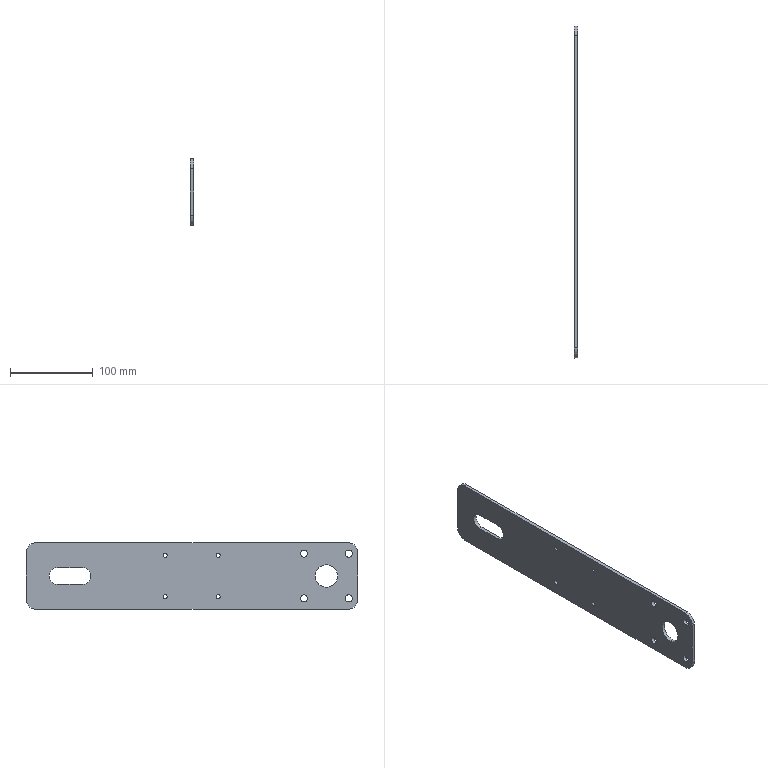Component | SolidWorks | BeltLineSidePlate-3_YL1.sldasm-Part-90-1 | 1 solid | 32 faces | box 4 x 400 x 80 mm | volume 120337 mm3 | cylinder 24 | plane 8 | commonest cylinder face diameters 5 x8 8.5 x8 24 x4 27 x2 20 x2
STEP:
#1=CARTESIAN_POINT('',(227.52,115.275,0.7825));
#2=VERTEX_POINT('',#1);
#3=CARTESIAN_POINT('',(227.52,115.275,0.9793));
#4=VERTEX_POINT('',#3);
#5=CARTESIAN_POINT('',(227.52,115.275,0.8809));
#6=DIRECTION('',(-1.,-0.,-0.));
#7=DIRECTION('',(0.,0.,1.));
#8=AXIS2_PLACEMENT_3D('',#5,#6,#7);
#9=CIRCLE('',#8,0.09843);
#10=EDGE_CURVE('',#2,#4,#9,.T.);
#11=ORIENTED_EDGE('',*,*,#10,.F.);
#12=CARTESIAN_POINT('',(227.362,115.275,0.7825));
#13=VERTEX_POINT('',#12);
#14=CARTESIAN_POINT('',(227.205,115.275,0.7825));
#15=DIRECTION('',(-1.,-0.,-0.));
#16=VECTOR('',#15,39.37);
#17=LINE('',#14,#16);
#18=EDGE_CURVE('',#2,#13,#17,.T.);
#19=ORIENTED_EDGE('',*,*,#18,.T.);
#20=CARTESIAN_POINT('',(227.362,115.275,0.9793));
#21=VERTEX_POINT('',#20);
#22=CARTESIAN_POINT('',(227.362,115.275,0.8809));
#23=DIRECTION('',(1.,0.,-0.));
#24=DIRECTION('',(0.,-1.,0.));
#25=AXIS2_PLACEMENT_3D('',#22,#23,#24);
#26=CIRCLE('',#25,0.09843);
#27=EDGE_CURVE('',#21,#13,#26,.T.);
#28=ORIENTED_EDGE('',*,*,#27,.F.);
#29=CARTESIAN_POINT('',(227.205,115.275,0.9793));
#30=DIRECTION('',(-1.,-0.,-0.));
#31=VECTOR('',#30,39.37);
#32=LINE('',#29,#31);
#33=EDGE_CURVE('',#4,#21,#32,.T.);
#34=ORIENTED_EDGE('',*,*,#33,.F.);
#35=EDGE_LOOP('',(#11,#19,#28,#34));
#36=FACE_OUTER_BOUND('',#35,.T.);
#37=CARTESIAN_POINT('',(227.205,115.275,0.8809));
#38=DIRECTION('',(-1.,-0.,-0.));
#39=DIRECTION('',(0.,0.,1.));
#40=AXIS2_PLACEMENT_3D('',#37,#38,#39);
#41=CYLINDRICAL_SURFACE('',#40,0.09843);
#42=ADVANCED_FACE('',(#36),#41,.F.);
#43=CARTESIAN_POINT('',(227.52,115.275,2.751));
#44=VERTEX_POINT('',#43);
#45=CARTESIAN_POINT('',(227.52,115.275,2.948));
#46=VERTEX_POINT('',#45);
#47=CARTESIAN_POINT('',(227.52,115.275,2.849));
#48=DIRECTION('',(-1.,-0.,-0.));
#49=DIRECTION('',(0.,0.,1.));
#50=AXIS2_PLACEMENT_3D('',#47,#48,#49);
#51=CIRCLE('',#50,0.09843);
#52=EDGE_CURVE('',#44,#46,#51,.T.);
#53=ORIENTED_EDGE('',*,*,#52,.F.);
#54=CARTESIAN_POINT('',(227.362,115.275,2.751));
#55=VERTEX_POINT('',#54);
#56=CARTESIAN_POINT('',(227.205,115.275,2.751));
#57=DIRECTION('',(-1.,-0.,-0.));
#58=VECTOR('',#57,39.37);
#59=LINE('',#56,#58);
#60=EDGE_CURVE('',#44,#55,#59,.T.);
#61=ORIENTED_EDGE('',*,*,#60,.T.);
#62=CARTESIAN_POINT('',(227.362,115.275,2.948));
#63=VERTEX_POINT('',#62);
#64=CARTESIAN_POINT('',(227.362,115.275,2.849));
#65=DIRECTION('',(1.,0.,-0.));
#66=DIRECTION('',(0.,-1.,0.));
#67=AXIS2_PLACEMENT_3D('',#64,#65,#66);
#68=CIRCLE('',#67,0.09843);
#69=EDGE_CURVE('',#63,#55,#68,.T.);
#70=ORIENTED_EDGE('',*,*,#69,.F.);
#71=CARTESIAN_POINT('',(227.205,115.275,2.948));
#72=DIRECTION('',(-1.,-0.,-0.));
#73=VECTOR('',#72,39.37);
#74=LINE('',#71,#73);
#75=EDGE_CURVE('',#46,#63,#74,.T.);
#76=ORIENTED_EDGE('',*,*,#75,.F.);
#77=EDGE_LOOP('',(#53,#61,#70,#76));
#78=FACE_OUTER_BOUND('',#77,.T.);
#79=CARTESIAN_POINT('',(227.205,115.275,2.849));
#80=DIRECTION('',(-1.,-0.,-0.));
#81=DIRECTION('',(0.,0.,1.));
#82=AXIS2_PLACEMENT_3D('',#79,#80,#81);
#83=CYLINDRICAL_SURFACE('',#82,0.09843);
#84=ADVANCED_FACE('',(#78),#83,.F.);
#85=CARTESIAN_POINT('',(227.52,112.756,0.7825));
#86=VERTEX_POINT('',#85);
#87=CARTESIAN_POINT('',(227.52,112.756,0.9793));
#88=VERTEX_POINT('',#87);
#89=CARTESIAN_POINT('',(227.52,112.756,0.8809));
#90=DIRECTION('',(-1.,-0.,-0.));
#91=DIRECTION('',(0.,0.,1.));
#92=AXIS2_PLACEMENT_3D('',#89,#90,#91);
#93=CIRCLE('',#92,0.09843);
#94=EDGE_CURVE('',#86,#88,#93,.T.);
#95=ORIENTED_EDGE('',*,*,#94,.F.);
#96=CARTESIAN_POINT('',(227.362,112.756,0.7825));
#97=VERTEX_POINT('',#96);
#98=CARTESIAN_POINT('',(227.205,112.756,0.7825));
#99=DIRECTION('',(-1.,-0.,-0.));
#100=VECTOR('',#99,39.37);
#101=LINE('',#98,#100);
#102=EDGE_CURVE('',#86,#97,#101,.T.);
#103=ORIENTED_EDGE('',*,*,#102,.T.);
#104=CARTESIAN_POINT('',(227.362,112.756,0.9793));
#105=VERTEX_POINT('',#104);
#106=CARTESIAN_POINT('',(227.362,112.756,0.8809));
#107=DIRECTION('',(1.,0.,-0.));
#108=DIRECTION('',(0.,-1.,0.));
#109=AXIS2_PLACEMENT_3D('',#106,#107,#108);
#110=CIRCLE('',#109,0.09843);
#111=EDGE_CURVE('',#105,#97,#110,.T.);
#112=ORIENTED_EDGE('',*,*,#111,.F.);
#113=CARTESIAN_POINT('',(227.205,112.756,0.9793));
#114=DIRECTION('',(-1.,-0.,-0.));
#115=VECTOR('',#114,39.37);
#116=LINE('',#113,#115);
#117=EDGE_CURVE('',#88,#105,#116,.T.);
#118=ORIENTED_EDGE('',*,*,#117,.F.);
#119=EDGE_LOOP('',(#95,#103,#112,#118));
#120=FACE_OUTER_BOUND('',#119,.T.);
#121=CARTESIAN_POINT('',(227.205,112.756,0.8809));
#122=DIRECTION('',(-1.,-0.,-0.));
#123=DIRECTION('',(0.,0.,1.));
#124=AXIS2_PLACEMENT_3D('',#121,#122,#123);
#125=CYLINDRICAL_SURFACE('',#124,0.09843);
#126=ADVANCED_FACE('',(#120),#125,.F.);
#127=CARTESIAN_POINT('',(227.52,112.756,2.751));
#128=VERTEX_POINT('',#127);
#129=CARTESIAN_POINT('',(227.52,112.756,2.948));
#130=VERTEX_POINT('',#129);
#131=CARTESIAN_POINT('',(227.52,112.756,2.849));
#132=DIRECTION('',(-1.,-0.,-0.));
#133=DIRECTION('',(0.,0.,1.));
#134=AXIS2_PLACEMENT_3D('',#131,#132,#133);
#135=CIRCLE('',#134,0.09843);
#136=EDGE_CURVE('',#128,#130,#135,.T.);
#137=ORIENTED_EDGE('',*,*,#136,.F.);
#138=CARTESIAN_POINT('',(227.362,112.756,2.751));
#139=VERTEX_POINT('',#138);
#140=CARTESIAN_POINT('',(227.205,112.756,2.751));
#141=DIRECTION('',(-1.,-0.,-0.));
#142=VECTOR('',#141,39.37);
#143=LINE('',#140,#142);
#144=EDGE_CURVE('',#128,#139,#143,.T.);
#145=ORIENTED_EDGE('',*,*,#144,.T.);
#146=CARTESIAN_POINT('',(227.362,112.756,2.948));
#147=VERTEX_POINT('',#146);
#148=CARTESIAN_POINT('',(227.362,112.756,2.849));
#149=DIRECTION('',(1.,0.,-0.));
#150=DIRECTION('',(0.,-1.,0.));
#151=AXIS2_PLACEMENT_3D('',#148,#149,#150);
#152=CIRCLE('',#151,0.09843);
#153=EDGE_CURVE('',#147,#139,#152,.T.);
#154=ORIENTED_EDGE('',*,*,#153,.F.);
#155=CARTESIAN_POINT('',(227.205,112.756,2.948));
#156=DIRECTION('',(-1.,-0.,-0.));
#157=VECTOR('',#156,39.37);
#158=LINE('',#155,#157);
#159=EDGE_CURVE('',#130,#147,#158,.T.);
#160=ORIENTED_EDGE('',*,*,#159,.F.);
#161=EDGE_LOOP('',(#137,#145,#154,#160));
#162=FACE_OUTER_BOUND('',#161,.T.);
#163=CARTESIAN_POINT('',(227.205,112.756,2.849));
#164=DIRECTION('',(-1.,-0.,-0.));
#165=DIRECTION('',(0.,0.,1.));
#166=AXIS2_PLACEMENT_3D('',#163,#164,#165);
#167=CYLINDRICAL_SURFACE('',#166,0.09843);
#168=ADVANCED_FACE('',(#162),#167,.F.);
#169=CARTESIAN_POINT('',(227.52,108.688,0.6348));
#170=VERTEX_POINT('',#169);
#171=CARTESIAN_POINT('',(227.52,108.688,0.9695));
#172=VERTEX_POINT('',#171);
#173=CARTESIAN_POINT('',(227.52,108.688,0.8022));
#174=DIRECTION('',(-1.,-0.,0.));
#175=DIRECTION('',(0.,0.,1.));
#176=AXIS2_PLACEMENT_3D('',#173,#174,#175);
#177=CIRCLE('',#176,0.1673);
#178=EDGE_CURVE('',#170,#172,#177,.T.);
#179=ORIENTED_EDGE('',*,*,#178,.F.);
#180=CARTESIAN_POINT('',(227.362,108.688,0.6348));
#181=VERTEX_POINT('',#180);
#182=CARTESIAN_POINT('',(227.362,108.688,0.6348));
#183=DIRECTION('',(-1.,-0.,0.));
#184=VECTOR('',#183,39.37);
#185=LINE('',#182,#184);
#186=EDGE_CURVE('',#170,#181,#185,.T.);
#187=ORIENTED_EDGE('',*,*,#186,.T.);
#188=CARTESIAN_POINT('',(227.362,108.688,0.9695));
#189=VERTEX_POINT('',#188);
#190=CARTESIAN_POINT('',(227.362,108.688,0.8022));
#191=DIRECTION('',(-1.,-0.,0.));
#192=DIRECTION('',(0.,0.,1.));
#193=AXIS2_PLACEMENT_3D('',#190,#191,#192);
#194=CIRCLE('',#193,0.1673);
#195=EDGE_CURVE('',#181,#189,#194,.T.);
#196=ORIENTED_EDGE('',*,*,#195,.T.);
#197=CARTESIAN_POINT('',(227.362,108.688,0.9695));
#198=DIRECTION('',(-1.,-0.,0.));
#199=VECTOR('',#198,39.37);
#200=LINE('',#197,#199);
#201=EDGE_CURVE('',#172,#189,#200,.T.);
#202=ORIENTED_EDGE('',*,*,#201,.F.);
#203=EDGE_LOOP('',(#179,#187,#196,#202));
#204=FACE_OUTER_BOUND('',#203,.T.);
#205=CARTESIAN_POINT('',(227.362,108.688,0.8022));
#206=DIRECTION('',(-1.,-0.,0.));
#207=DIRECTION('',(0.,0.,1.));
#208=AXIS2_PLACEMENT_3D('',#205,#206,#207);
#209=CYLINDRICAL_SURFACE('',#208,0.1673);
#210=ADVANCED_FACE('',(#204),#209,.F.);
#211=CARTESIAN_POINT('',(227.52,108.688,2.761));
#212=VERTEX_POINT('',#211);
#213=CARTESIAN_POINT('',(227.52,108.688,3.095));
#214=VERTEX_POINT('',#213);
#215=CARTESIAN_POINT('',(227.52,108.688,2.928));
#216=DIRECTION('',(-1.,-0.,0.));
#217=DIRECTION('',(0.,0.,1.));
#218=AXIS2_PLACEMENT_3D('',#215,#216,#217);
#219=CIRCLE('',#218,0.1673);
#220=EDGE_CURVE('',#212,#214,#219,.T.);
#221=ORIENTED_EDGE('',*,*,#220,.F.);
#222=CARTESIAN_POINT('',(227.362,108.688,2.761));
#223=VERTEX_POINT('',#222);
#224=CARTESIAN_POINT('',(227.362,108.688,2.761));
#225=DIRECTION('',(-1.,-0.,0.));
#226=VECTOR('',#225,39.37);
#227=LINE('',#224,#226);
#228=EDGE_CURVE('',#212,#223,#227,.T.);
#229=ORIENTED_EDGE('',*,*,#228,.T.);
#230=CARTESIAN_POINT('',(227.362,108.688,3.095));
#231=VERTEX_POINT('',#230);
#232=CARTESIAN_POINT('',(227.362,108.688,2.928));
#233=DIRECTION('',(-1.,-0.,0.));
#234=DIRECTION('',(0.,0.,1.));
#235=AXIS2_PLACEMENT_3D('',#232,#233,#234);
#236=CIRCLE('',#235,0.1673);
#237=EDGE_CURVE('',#223,#231,#236,.T.);
#238=ORIENTED_EDGE('',*,*,#237,.T.);
#239=CARTESIAN_POINT('',(227.362,108.688,3.095));
#240=DIRECTION('',(-1.,-0.,0.));
#241=VECTOR('',#240,39.37);
#242=LINE('',#239,#241);
#243=EDGE_CURVE('',#214,#231,#242,.T.);
#244=ORIENTED_EDGE('',*,*,#243,.F.);
#245=EDGE_LOOP('',(#221,#229,#238,#244));
#246=FACE_OUTER_BOUND('',#245,.T.);
#247=CARTESIAN_POINT('',(227.362,108.688,2.928));
#248=DIRECTION('',(-1.,-0.,0.));
#249=DIRECTION('',(0.,0.,1.));
#250=AXIS2_PLACEMENT_3D('',#247,#248,#249);
#251=CYLINDRICAL_SURFACE('',#250,0.1673);
#252=ADVANCED_FACE('',(#246),#251,.F.);
#253=CARTESIAN_POINT('',(227.52,106.562,0.6348));
#254=VERTEX_POINT('',#253);
#255=CARTESIAN_POINT('',(227.52,106.562,0.9695));
#256=VERTEX_POINT('',#255);
#257=CARTESIAN_POINT('',(227.52,106.562,0.8022));
#258=DIRECTION('',(-1.,-0.,0.));
#259=DIRECTION('',(0.,0.,1.));
#260=AXIS2_PLACEMENT_3D('',#257,#258,#259);
#261=CIRCLE('',#260,0.1673);
#262=EDGE_CURVE('',#254,#256,#261,.T.);
#263=ORIENTED_EDGE('',*,*,#262,.F.);
#264=CARTESIAN_POINT('',(227.362,106.562,0.6348));
#265=VERTEX_POINT('',#264);
#266=CARTESIAN_POINT('',(227.362,106.562,0.6348));
#267=DIRECTION('',(-1.,-0.,0.));
#268=VECTOR('',#267,39.37);
#269=LINE('',#266,#268);
#270=EDGE_CURVE('',#254,#265,#269,.T.);
#271=ORIENTED_EDGE('',*,*,#270,.T.);
#272=CARTESIAN_POINT('',(227.362,106.562,0.9695));
#273=VERTEX_POINT('',#272);
#274=CARTESIAN_POINT('',(227.362,106.562,0.8022));
#275=DIRECTION('',(-1.,-0.,0.));
#276=DIRECTION('',(0.,0.,1.));
#277=AXIS2_PLACEMENT_3D('',#274,#275,#276);
#278=CIRCLE('',#277,0.1673);
#279=EDGE_CURVE('',#265,#273,#278,.T.);
#280=ORIENTED_EDGE('',*,*,#279,.T.);
#281=CARTESIAN_POINT('',(227.362,106.562,0.9695));
#282=DIRECTION('',(-1.,-0.,0.));
#283=VECTOR('',#282,39.37);
#284=LINE('',#281,#283);
#285=EDGE_CURVE('',#256,#273,#284,.T.);
#286=ORIENTED_EDGE('',*,*,#285,.F.);
#287=EDGE_LOOP('',(#263,#271,#280,#286));
#288=FACE_OUTER_BOUND('',#287,.T.);
#289=CARTESIAN_POINT('',(227.362,106.562,0.8022));
#290=DIRECTION('',(-1.,-0.,0.));
#291=DIRECTION('',(0.,0.,1.));
#292=AXIS2_PLACEMENT_3D('',#289,#290,#291);
#293=CYLINDRICAL_SURFACE('',#292,0.1673);
#294=ADVANCED_FACE('',(#288),#293,.F.);
#295=CARTESIAN_POINT('',(227.52,106.562,2.761));
#296=VERTEX_POINT('',#295);
#297=CARTESIAN_POINT('',(227.52,106.562,3.095));
#298=VERTEX_POINT('',#297);
#299=CARTESIAN_POINT('',(227.52,106.562,2.928));
#300=DIRECTION('',(-1.,-0.,0.));
#301=DIRECTION('',(0.,0.,1.));
#302=AXIS2_PLACEMENT_3D('',#299,#300,#301);
#303=CIRCLE('',#302,0.1673);
#304=EDGE_CURVE('',#296,#298,#303,.T.);
#305=ORIENTED_EDGE('',*,*,#304,.F.);
#306=CARTESIAN_POINT('',(227.362,106.562,2.761));
#307=VERTEX_POINT('',#306);
#308=CARTESIAN_POINT('',(227.362,106.562,2.761));
#309=DIRECTION('',(-1.,-0.,0.));
#310=VECTOR('',#309,39.37);
#311=LINE('',#308,#310);
#312=EDGE_CURVE('',#296,#307,#311,.T.);
#313=ORIENTED_EDGE('',*,*,#312,.T.);
#314=CARTESIAN_POINT('',(227.362,106.562,3.095));
#315=VERTEX_POINT('',#314);
#316=CARTESIAN_POINT('',(227.362,106.562,2.928));
#317=DIRECTION('',(-1.,-0.,0.));
#318=DIRECTION('',(0.,0.,1.));
#319=AXIS2_PLACEMENT_3D('',#316,#317,#318);
#320=CIRCLE('',#319,0.1673);
#321=EDGE_CURVE('',#307,#315,#320,.T.);
#322=ORIENTED_EDGE('',*,*,#321,.T.);
#323=CARTESIAN_POINT('',(227.362,106.562,3.095));
#324=DIRECTION('',(-1.,-0.,0.));
#325=VECTOR('',#324,39.37);
#326=LINE('',#323,#325);
#327=EDGE_CURVE('',#298,#315,#326,.T.);
#328=ORIENTED_EDGE('',*,*,#327,.F.);
#329=EDGE_LOOP('',(#305,#313,#322,#328));
#330=FACE_OUTER_BOUND('',#329,.T.);
#331=CARTESIAN_POINT('',(227.362,106.562,2.928));
#332=DIRECTION('',(-1.,-0.,0.));
#333=DIRECTION('',(0.,0.,1.));
#334=AXIS2_PLACEMENT_3D('',#331,#332,#333);
#335=CYLINDRICAL_SURFACE('',#334,0.1673);
#336=ADVANCED_FACE('',(#330),#335,.F.);
#337=CARTESIAN_POINT('',(227.52,107.625,1.334));
#338=VERTEX_POINT('',#337);
#339=CARTESIAN_POINT('',(227.52,107.625,2.397));
#340=VERTEX_POINT('',#339);
#341=CARTESIAN_POINT('',(227.52,107.625,1.865));
#342=DIRECTION('',(-1.,-0.,0.));
#343=DIRECTION('',(0.,0.,1.));
#344=AXIS2_PLACEMENT_3D('',#341,#342,#343);
#345=CIRCLE('',#344,0.5315);
#346=EDGE_CURVE('',#338,#340,#345,.T.);
#347=ORIENTED_EDGE('',*,*,#346,.F.);
#348=CARTESIAN_POINT('',(227.362,107.625,1.334));
#349=VERTEX_POINT('',#348);
#350=CARTESIAN_POINT('',(229.154,107.625,1.334));
#351=DIRECTION('',(-1.,-0.,-0.));
#352=VECTOR('',#351,39.37);
#353=LINE('',#350,#352);
#354=EDGE_CURVE('',#338,#349,#353,.T.);
#355=ORIENTED_EDGE('',*,*,#354,.T.);
#356=CARTESIAN_POINT('',(227.362,107.625,2.397));
#357=VERTEX_POINT('',#356);
#358=CARTESIAN_POINT('',(227.362,107.625,1.865));
#359=DIRECTION('',(1.,0.,-0.));
#360=DIRECTION('',(0.,0.,-1.));
#361=AXIS2_PLACEMENT_3D('',#358,#359,#360);
#362=CIRCLE('',#361,0.5315);
#363=EDGE_CURVE('',#357,#349,#362,.T.);
#364=ORIENTED_EDGE('',*,*,#363,.F.);
#365=CARTESIAN_POINT('',(229.154,107.625,2.397));
#366=DIRECTION('',(-1.,-0.,-0.));
#367=VECTOR('',#366,39.37);
#368=LINE('',#365,#367);
#369=EDGE_CURVE('',#340,#357,#368,.T.);
#370=ORIENTED_EDGE('',*,*,#369,.F.);
#371=EDGE_LOOP('',(#347,#355,#364,#370));
#372=FACE_OUTER_BOUND('',#371,.T.);
#373=CARTESIAN_POINT('',(229.154,107.625,1.865));
#374=DIRECTION('',(-1.,-0.,-0.));
#375=DIRECTION('',(0.,0.,1.));
#376=AXIS2_PLACEMENT_3D('',#373,#374,#375);
#377=CYLINDRICAL_SURFACE('',#376,0.5315);
#378=ADVANCED_FACE('',(#372),#377,.F.);
#379=ORIENTED_EDGE('',*,*,#27,.T.);
#380=CARTESIAN_POINT('',(227.362,115.275,0.8809));
#381=DIRECTION('',(1.,0.,-0.));
#382=DIRECTION('',(0.,-1.,0.));
#383=AXIS2_PLACEMENT_3D('',#380,#381,#382);
#384=CIRCLE('',#383,0.09843);
#385=EDGE_CURVE('',#13,#21,#384,.T.);
#386=ORIENTED_EDGE('',*,*,#385,.T.);
#387=EDGE_LOOP('',(#379,#386));
#388=FACE_BOUND('',#387,.T.);
#389=ORIENTED_EDGE('',*,*,#69,.T.);
#390=CARTESIAN_POINT('',(227.362,115.275,2.849));
#391=DIRECTION('',(1.,0.,-0.));
#392=DIRECTION('',(0.,-1.,0.));
#393=AXIS2_PLACEMENT_3D('',#390,#391,#392);
#394=CIRCLE('',#393,0.09843);
#395=EDGE_CURVE('',#55,#63,#394,.T.);
#396=ORIENTED_EDGE('',*,*,#395,.T.);
#397=EDGE_LOOP('',(#389,#396));
#398=FACE_BOUND('',#397,.T.);
#399=ORIENTED_EDGE('',*,*,#111,.T.);
#400=CARTESIAN_POINT('',(227.362,112.756,0.8809));
#401=DIRECTION('',(1.,0.,-0.));
#402=DIRECTION('',(0.,-1.,0.));
#403=AXIS2_PLACEMENT_3D('',#400,#401,#402);
#404=CIRCLE('',#403,0.09843);
#405=EDGE_CURVE('',#97,#105,#404,.T.);
#406=ORIENTED_EDGE('',*,*,#405,.T.);
#407=EDGE_LOOP('',(#399,#406));
#408=FACE_BOUND('',#407,.T.);
#409=ORIENTED_EDGE('',*,*,#153,.T.);
#410=CARTESIAN_POINT('',(227.362,112.756,2.849));
#411=DIRECTION('',(1.,0.,-0.));
#412=DIRECTION('',(0.,-1.,0.));
#413=AXIS2_PLACEMENT_3D('',#410,#411,#412);
#414=CIRCLE('',#413,0.09843);
#415=EDGE_CURVE('',#139,#147,#414,.T.);
#416=ORIENTED_EDGE('',*,*,#415,.T.);
#417=EDGE_LOOP('',(#409,#416));
#418=FACE_BOUND('',#417,.T.);
#419=CARTESIAN_POINT('',(227.362,108.688,0.8022));
#420=DIRECTION('',(-1.,-0.,0.));
#421=DIRECTION('',(0.,0.,1.));
#422=AXIS2_PLACEMENT_3D('',#419,#420,#421);
#423=CIRCLE('',#422,0.1673);
#424=EDGE_CURVE('',#189,#181,#423,.T.);
#425=ORIENTED_EDGE('',*,*,#424,.F.);
#426=ORIENTED_EDGE('',*,*,#195,.F.);
#427=EDGE_LOOP('',(#425,#426));
#428=FACE_BOUND('',#427,.T.);
#429=CARTESIAN_POINT('',(227.362,108.688,2.928));
#430=DIRECTION('',(-1.,-0.,0.));
#431=DIRECTION('',(0.,0.,1.));
#432=AXIS2_PLACEMENT_3D('',#429,#430,#431);
#433=CIRCLE('',#432,0.1673);
#434=EDGE_CURVE('',#231,#223,#433,.T.);
#435=ORIENTED_EDGE('',*,*,#434,.F.);
#436=ORIENTED_EDGE('',*,*,#237,.F.);
#437=EDGE_LOOP('',(#435,#436));
#438=FACE_BOUND('',#437,.T.);
#439=CARTESIAN_POINT('',(227.362,106.562,0.8022));
#440=DIRECTION('',(-1.,-0.,0.));
#441=DIRECTION('',(0.,0.,1.));
#442=AXIS2_PLACEMENT_3D('',#439,#440,#441);
#443=CIRCLE('',#442,0.1673);
#444=EDGE_CURVE('',#273,#265,#443,.T.);
#445=ORIENTED_EDGE('',*,*,#444,.F.);
#446=ORIENTED_EDGE('',*,*,#279,.F.);
#447=EDGE_LOOP('',(#445,#446));
#448=FACE_BOUND('',#447,.T.);
#449=CARTESIAN_POINT('',(227.362,106.562,2.928));
#450=DIRECTION('',(-1.,-0.,0.));
#451=DIRECTION('',(0.,0.,1.));
#452=AXIS2_PLACEMENT_3D('',#449,#450,#451);
#453=CIRCLE('',#452,0.1673);
#454=EDGE_CURVE('',#315,#307,#453,.T.);
#455=ORIENTED_EDGE('',*,*,#454,.F.);
#456=ORIENTED_EDGE('',*,*,#321,.F.);
#457=EDGE_LOOP('',(#455,#456));
#458=FACE_BOUND('',#457,.T.);
#459=ORIENTED_EDGE('',*,*,#363,.T.);
#460=CARTESIAN_POINT('',(227.362,107.625,1.865));
#461=DIRECTION('',(1.,0.,-0.));
#462=DIRECTION('',(0.,0.,-1.));
#463=AXIS2_PLACEMENT_3D('',#460,#461,#462);
#464=CIRCLE('',#463,0.5315);
#465=EDGE_CURVE('',#349,#357,#464,.T.);
#466=ORIENTED_EDGE('',*,*,#465,.T.);
#467=EDGE_LOOP('',(#459,#466));
#468=FACE_BOUND('',#467,.T.);
#469=CARTESIAN_POINT('',(227.362,121.405,3.44));
#470=VERTEX_POINT('',#469);
#471=CARTESIAN_POINT('',(227.362,106.602,3.44));
#472=VERTEX_POINT('',#471);
#473=CARTESIAN_POINT('',(227.362,184.869,3.44));
#474=DIRECTION('',(0.,-1.,0.));
#475=VECTOR('',#474,39.37);
#476=LINE('',#473,#475);
#477=EDGE_CURVE('',#470,#472,#476,.T.);
#478=ORIENTED_EDGE('',*,*,#477,.F.);
#479=CARTESIAN_POINT('',(227.362,121.877,2.968));
#480=VERTEX_POINT('',#479);
#481=CARTESIAN_POINT('',(227.362,121.405,2.968));
#482=DIRECTION('',(-1.,-0.,0.));
#483=DIRECTION('',(0.,0.,-1.));
#484=AXIS2_PLACEMENT_3D('',#481,#482,#483);
#485=CIRCLE('',#484,0.4724);
#486=EDGE_CURVE('',#470,#480,#485,.T.);
#487=ORIENTED_EDGE('',*,*,#486,.T.);
#488=CARTESIAN_POINT('',(227.362,121.877,0.7628));
#489=VERTEX_POINT('',#488);
#490=CARTESIAN_POINT('',(227.362,121.877,0.3691));
#491=DIRECTION('',(0.,0.,1.));
#492=VECTOR('',#491,39.37);
#493=LINE('',#490,#492);
#494=EDGE_CURVE('',#489,#480,#493,.T.);
#495=ORIENTED_EDGE('',*,*,#494,.F.);
#496=CARTESIAN_POINT('',(227.362,121.405,0.2904));
#497=VERTEX_POINT('',#496);
#498=CARTESIAN_POINT('',(227.362,121.405,0.7628));
#499=DIRECTION('',(-1.,-0.,0.));
#500=DIRECTION('',(0.,0.,-1.));
#501=AXIS2_PLACEMENT_3D('',#498,#499,#500);
#502=CIRCLE('',#501,0.4724);
#503=EDGE_CURVE('',#489,#497,#502,.T.);
#504=ORIENTED_EDGE('',*,*,#503,.T.);
#505=CARTESIAN_POINT('',(227.362,106.602,0.2904));
#506=VERTEX_POINT('',#505);
#507=CARTESIAN_POINT('',(227.362,184.869,0.2904));
#508=DIRECTION('',(0.,-1.,0.));
#509=VECTOR('',#508,39.37);
#510=LINE('',#507,#509);
#511=EDGE_CURVE('',#497,#506,#510,.T.);
#512=ORIENTED_EDGE('',*,*,#511,.T.);
#513=CARTESIAN_POINT('',(227.362,106.129,0.7628));
#514=VERTEX_POINT('',#513);
#515=CARTESIAN_POINT('',(227.362,106.602,0.7628));
#516=DIRECTION('',(-1.,-0.,0.));
#517=DIRECTION('',(0.,0.,-1.));
#518=AXIS2_PLACEMENT_3D('',#515,#516,#517);
#519=CIRCLE('',#518,0.4724);
#520=EDGE_CURVE('',#506,#514,#519,.T.);
#521=ORIENTED_EDGE('',*,*,#520,.T.);
#522=CARTESIAN_POINT('',(227.362,106.129,2.968));
#523=VERTEX_POINT('',#522);
#524=CARTESIAN_POINT('',(227.362,106.129,0.3691));
#525=DIRECTION('',(0.,0.,1.));
#526=VECTOR('',#525,39.37);
#527=LINE('',#524,#526);
#528=EDGE_CURVE('',#514,#523,#527,.T.);
#529=ORIENTED_EDGE('',*,*,#528,.T.);
#530=CARTESIAN_POINT('',(227.362,106.602,2.968));
#531=DIRECTION('',(-1.,-0.,0.));
#532=DIRECTION('',(0.,0.,-1.));
#533=AXIS2_PLACEMENT_3D('',#530,#531,#532);
#534=CIRCLE('',#533,0.4724);
#535=EDGE_CURVE('',#523,#472,#534,.T.);
#536=ORIENTED_EDGE('',*,*,#535,.T.);
#537=EDGE_LOOP('',(#478,#487,#495,#504,#512,#521,#529,#536));
#538=FACE_OUTER_BOUND('',#537,.T.);
#539=CARTESIAN_POINT('',(227.362,120.381,1.471));
#540=VERTEX_POINT('',#539);
#541=CARTESIAN_POINT('',(227.362,119.2,1.471));
#542=VERTEX_POINT('',#541);
#543=CARTESIAN_POINT('',(227.362,121.877,1.471));
#544=DIRECTION('',(0.,-1.,0.));
#545=VECTOR('',#544,39.37);
#546=LINE('',#543,#545);
#547=EDGE_CURVE('',#540,#542,#546,.T.);
#548=ORIENTED_EDGE('',*,*,#547,.F.);
#549=CARTESIAN_POINT('',(227.362,120.381,2.259));
#550=VERTEX_POINT('',#549);
#551=CARTESIAN_POINT('',(227.362,120.381,1.865));
#552=DIRECTION('',(-1.,-0.,0.));
#553=DIRECTION('',(0.,0.,-1.));
#554=AXIS2_PLACEMENT_3D('',#551,#552,#553);
#555=CIRCLE('',#554,0.3937);
#556=EDGE_CURVE('',#550,#540,#555,.T.);
#557=ORIENTED_EDGE('',*,*,#556,.F.);
#558=CARTESIAN_POINT('',(227.362,119.2,2.259));
#559=VERTEX_POINT('',#558);
#560=CARTESIAN_POINT('',(227.362,121.877,2.259));
#561=DIRECTION('',(-0.,1.,0.));
#562=VECTOR('',#561,39.37);
#563=LINE('',#560,#562);
#564=EDGE_CURVE('',#559,#550,#563,.T.);
#565=ORIENTED_EDGE('',*,*,#564,.F.);
#566=CARTESIAN_POINT('',(227.362,119.2,1.865));
#567=DIRECTION('',(-1.,-0.,0.));
#568=DIRECTION('',(0.,0.,-1.));
#569=AXIS2_PLACEMENT_3D('',#566,#567,#568);
#570=CIRCLE('',#569,0.3937);
#571=EDGE_CURVE('',#542,#559,#570,.T.);
#572=ORIENTED_EDGE('',*,*,#571,.F.);
#573=EDGE_LOOP('',(#548,#557,#565,#572));
#574=FACE_BOUND('',#573,.T.);
#575=CARTESIAN_POINT('',(227.362,184.869,0.3691));
#576=DIRECTION('',(1.,0.,-0.));
#577=DIRECTION('',(-0.,-0.,-1.));
#578=AXIS2_PLACEMENT_3D('',#575,#576,#577);
#579=PLANE('',#578);
#580=ADVANCED_FACE('',(#388,#398,#408,#418,#428,#438,#448,#458,#468,#538,#574),#579,.F.);
#581=CARTESIAN_POINT('',(227.52,115.275,0.8809));
#582=DIRECTION('',(-1.,-0.,-0.));
#583=DIRECTION('',(0.,0.,1.));
#584=AXIS2_PLACEMENT_3D('',#581,#582,#583);
#585=CIRCLE('',#584,0.09843);
#586=EDGE_CURVE('',#4,#2,#585,.T.);
#587=ORIENTED_EDGE('',*,*,#586,.T.);
#588=ORIENTED_EDGE('',*,*,#10,.T.);
#589=EDGE_LOOP('',(#587,#588));
#590=FACE_BOUND('',#589,.T.);
#591=CARTESIAN_POINT('',(227.52,115.275,2.849));
#592=DIRECTION('',(-1.,-0.,-0.));
#593=DIRECTION('',(0.,0.,1.));
#594=AXIS2_PLACEMENT_3D('',#591,#592,#593);
#595=CIRCLE('',#594,0.09843);
#596=EDGE_CURVE('',#46,#44,#595,.T.);
#597=ORIENTED_EDGE('',*,*,#596,.T.);
#598=ORIENTED_EDGE('',*,*,#52,.T.);
#599=EDGE_LOOP('',(#597,#598));
#600=FACE_BOUND('',#599,.T.);
#601=CARTESIAN_POINT('',(227.52,112.756,0.8809));
#602=DIRECTION('',(-1.,-0.,-0.));
#603=DIRECTION('',(0.,0.,1.));
#604=AXIS2_PLACEMENT_3D('',#601,#602,#603);
#605=CIRCLE('',#604,0.09843);
#606=EDGE_CURVE('',#88,#86,#605,.T.);
#607=ORIENTED_EDGE('',*,*,#606,.T.);
#608=ORIENTED_EDGE('',*,*,#94,.T.);
#609=EDGE_LOOP('',(#607,#608));
#610=FACE_BOUND('',#609,.T.);
#611=CARTESIAN_POINT('',(227.52,112.756,2.849));
#612=DIRECTION('',(-1.,-0.,-0.));
#613=DIRECTION('',(0.,0.,1.));
#614=AXIS2_PLACEMENT_3D('',#611,#612,#613);
#615=CIRCLE('',#614,0.09843);
#616=EDGE_CURVE('',#130,#128,#615,.T.);
#617=ORIENTED_EDGE('',*,*,#616,.T.);
#618=ORIENTED_EDGE('',*,*,#136,.T.);
#619=EDGE_LOOP('',(#617,#618));
#620=FACE_BOUND('',#619,.T.);
#621=CARTESIAN_POINT('',(227.52,108.688,0.8022));
#622=DIRECTION('',(-1.,-0.,0.));
#623=DIRECTION('',(0.,0.,1.));
#624=AXIS2_PLACEMENT_3D('',#621,#622,#623);
#625=CIRCLE('',#624,0.1673);
#626=EDGE_CURVE('',#172,#170,#625,.T.);
#627=ORIENTED_EDGE('',*,*,#626,.T.);
#628=ORIENTED_EDGE('',*,*,#178,.T.);
#629=EDGE_LOOP('',(#627,#628));
#630=FACE_BOUND('',#629,.T.);
#631=CARTESIAN_POINT('',(227.52,108.688,2.928));
#632=DIRECTION('',(-1.,-0.,0.));
#633=DIRECTION('',(0.,0.,1.));
#634=AXIS2_PLACEMENT_3D('',#631,#632,#633);
#635=CIRCLE('',#634,0.1673);
#636=EDGE_CURVE('',#214,#212,#635,.T.);
#637=ORIENTED_EDGE('',*,*,#636,.T.);
#638=ORIENTED_EDGE('',*,*,#220,.T.);
#639=EDGE_LOOP('',(#637,#638));
#640=FACE_BOUND('',#639,.T.);
#641=CARTESIAN_POINT('',(227.52,106.562,0.8022));
#642=DIRECTION('',(-1.,-0.,0.));
#643=DIRECTION('',(0.,0.,1.));
#644=AXIS2_PLACEMENT_3D('',#641,#642,#643);
#645=CIRCLE('',#644,0.1673);
#646=EDGE_CURVE('',#256,#254,#645,.T.);
#647=ORIENTED_EDGE('',*,*,#646,.T.);
#648=ORIENTED_EDGE('',*,*,#262,.T.);
#649=EDGE_LOOP('',(#647,#648));
#650=FACE_BOUND('',#649,.T.);
#651=CARTESIAN_POINT('',(227.52,106.562,2.928));
#652=DIRECTION('',(-1.,-0.,0.));
#653=DIRECTION('',(0.,0.,1.));
#654=AXIS2_PLACEMENT_3D('',#651,#652,#653);
#655=CIRCLE('',#654,0.1673);
#656=EDGE_CURVE('',#298,#296,#655,.T.);
#657=ORIENTED_EDGE('',*,*,#656,.T.);
#658=ORIENTED_EDGE('',*,*,#304,.T.);
#659=EDGE_LOOP('',(#657,#658));
#660=FACE_BOUND('',#659,.T.);
#661=CARTESIAN_POINT('',(227.52,107.625,1.865));
#662=DIRECTION('',(-1.,-0.,0.));
#663=DIRECTION('',(0.,0.,1.));
#664=AXIS2_PLACEMENT_3D('',#661,#662,#663);
#665=CIRCLE('',#664,0.5315);
#666=EDGE_CURVE('',#340,#338,#665,.T.);
#667=ORIENTED_EDGE('',*,*,#666,.T.);
#668=ORIENTED_EDGE('',*,*,#346,.T.);
#669=EDGE_LOOP('',(#667,#668));
#670=FACE_BOUND('',#669,.T.);
#671=CARTESIAN_POINT('',(227.52,106.602,0.2904));
#672=VERTEX_POINT('',#671);
#673=CARTESIAN_POINT('',(227.52,121.405,0.2904));
#674=VERTEX_POINT('',#673);
#675=CARTESIAN_POINT('',(227.52,184.869,0.2904));
#676=DIRECTION('',(-0.,1.,-0.));
#677=VECTOR('',#676,39.37);
#678=LINE('',#675,#677);
#679=EDGE_CURVE('',#672,#674,#678,.T.);
#680=ORIENTED_EDGE('',*,*,#679,.T.);
#681=CARTESIAN_POINT('',(227.52,121.877,0.7628));
#682=VERTEX_POINT('',#681);
#683=CARTESIAN_POINT('',(227.52,121.405,0.7628));
#684=DIRECTION('',(1.,0.,-0.));
#685=DIRECTION('',(0.,0.,1.));
#686=AXIS2_PLACEMENT_3D('',#683,#684,#685);
#687=CIRCLE('',#686,0.4724);
#688=EDGE_CURVE('',#674,#682,#687,.T.);
#689=ORIENTED_EDGE('',*,*,#688,.T.);
#690=CARTESIAN_POINT('',(227.52,121.877,2.968));
#691=VERTEX_POINT('',#690);
#692=CARTESIAN_POINT('',(227.52,121.877,3.322));
#693=DIRECTION('',(-0.,-0.,-1.));
#694=VECTOR('',#693,39.37);
#695=LINE('',#692,#694);
#696=EDGE_CURVE('',#691,#682,#695,.T.);
#697=ORIENTED_EDGE('',*,*,#696,.F.);
#698=CARTESIAN_POINT('',(227.52,121.405,3.44));
#699=VERTEX_POINT('',#698);
#700=CARTESIAN_POINT('',(227.52,121.405,2.968));
#701=DIRECTION('',(1.,0.,-0.));
#702=DIRECTION('',(0.,0.,1.));
#703=AXIS2_PLACEMENT_3D('',#700,#701,#702);
#704=CIRCLE('',#703,0.4724);
#705=EDGE_CURVE('',#691,#699,#704,.T.);
#706=ORIENTED_EDGE('',*,*,#705,.T.);
#707=CARTESIAN_POINT('',(227.52,106.602,3.44));
#708=VERTEX_POINT('',#707);
#709=CARTESIAN_POINT('',(227.52,184.869,3.44));
#710=DIRECTION('',(0.,-1.,0.));
#711=VECTOR('',#710,39.37);
#712=LINE('',#709,#711);
#713=EDGE_CURVE('',#699,#708,#712,.T.);
#714=ORIENTED_EDGE('',*,*,#713,.T.);
#715=CARTESIAN_POINT('',(227.52,106.129,2.968));
#716=VERTEX_POINT('',#715);
#717=CARTESIAN_POINT('',(227.52,106.602,2.968));
#718=DIRECTION('',(1.,0.,-0.));
#719=DIRECTION('',(0.,0.,1.));
#720=AXIS2_PLACEMENT_3D('',#717,#718,#719);
#721=CIRCLE('',#720,0.4724);
#722=EDGE_CURVE('',#708,#716,#721,.T.);
#723=ORIENTED_EDGE('',*,*,#722,.T.);
#724=CARTESIAN_POINT('',(227.52,106.129,0.7628));
#725=VERTEX_POINT('',#724);
#726=CARTESIAN_POINT('',(227.52,106.129,3.322));
#727=DIRECTION('',(-0.,-0.,-1.));
#728=VECTOR('',#727,39.37);
#729=LINE('',#726,#728);
#730=EDGE_CURVE('',#716,#725,#729,.T.);
#731=ORIENTED_EDGE('',*,*,#730,.T.);
#732=CARTESIAN_POINT('',(227.52,106.602,0.7628));
#733=DIRECTION('',(1.,0.,-0.));
#734=DIRECTION('',(0.,0.,1.));
#735=AXIS2_PLACEMENT_3D('',#732,#733,#734);
#736=CIRCLE('',#735,0.4724);
#737=EDGE_CURVE('',#725,#672,#736,.T.);
#738=ORIENTED_EDGE('',*,*,#737,.T.);
#739=EDGE_LOOP('',(#680,#689,#697,#706,#714,#723,#731,#738));
#740=FACE_OUTER_BOUND('',#739,.T.);
#741=CARTESIAN_POINT('',(227.52,119.2,1.471));
#742=VERTEX_POINT('',#741);
#743=CARTESIAN_POINT('',(227.52,120.381,1.471));
#744=VERTEX_POINT('',#743);
#745=CARTESIAN_POINT('',(227.52,121.877,1.471));
#746=DIRECTION('',(-0.,1.,-0.));
#747=VECTOR('',#746,39.37);
#748=LINE('',#745,#747);
#749=EDGE_CURVE('',#742,#744,#748,.T.);
#750=ORIENTED_EDGE('',*,*,#749,.F.);
#751=CARTESIAN_POINT('',(227.52,119.2,2.259));
#752=VERTEX_POINT('',#751);
#753=CARTESIAN_POINT('',(227.52,119.2,1.865));
#754=DIRECTION('',(1.,0.,-0.));
#755=DIRECTION('',(0.,0.,1.));
#756=AXIS2_PLACEMENT_3D('',#753,#754,#755);
#757=CIRCLE('',#756,0.3937);
#758=EDGE_CURVE('',#752,#742,#757,.T.);
#759=ORIENTED_EDGE('',*,*,#758,.F.);
#760=CARTESIAN_POINT('',(227.52,120.381,2.259));
#761=VERTEX_POINT('',#760);
#762=CARTESIAN_POINT('',(227.52,121.877,2.259));
#763=DIRECTION('',(0.,-1.,-0.));
#764=VECTOR('',#763,39.37);
#765=LINE('',#762,#764);
#766=EDGE_CURVE('',#761,#752,#765,.T.);
#767=ORIENTED_EDGE('',*,*,#766,.F.);
#768=CARTESIAN_POINT('',(227.52,120.381,1.865));
#769=DIRECTION('',(1.,0.,-0.));
#770=DIRECTION('',(0.,0.,1.));
#771=AXIS2_PLACEMENT_3D('',#768,#769,#770);
#772=CIRCLE('',#771,0.3937);
#773=EDGE_CURVE('',#744,#761,#772,.T.);
#774=ORIENTED_EDGE('',*,*,#773,.F.);
#775=EDGE_LOOP('',(#750,#759,#767,#774));
#776=FACE_BOUND('',#775,.T.);
#777=CARTESIAN_POINT('',(227.52,184.869,3.322));
#778=DIRECTION('',(-1.,-0.,0.));
#779=DIRECTION('',(0.,0.,1.));
#780=AXIS2_PLACEMENT_3D('',#777,#778,#779);
#781=PLANE('',#780);
#782=ADVANCED_FACE('',(#590,#600,#610,#620,#630,#640,#650,#660,#670,#740,#776),#781,.F.);
#783=ORIENTED_EDGE('',*,*,#511,.F.);
#784=CARTESIAN_POINT('',(227.52,121.405,0.2904));
#785=DIRECTION('',(1.,0.,0.));
#786=VECTOR('',#785,39.37);
#787=LINE('',#784,#786);
#788=EDGE_CURVE('',#497,#674,#787,.T.);
#789=ORIENTED_EDGE('',*,*,#788,.T.);
#790=ORIENTED_EDGE('',*,*,#679,.F.);
#791=CARTESIAN_POINT('',(229.922,106.602,0.2904));
#792=DIRECTION('',(-1.,-0.,-0.));
#793=VECTOR('',#792,39.37);
#794=LINE('',#791,#793);
#795=EDGE_CURVE('',#672,#506,#794,.T.);
#796=ORIENTED_EDGE('',*,*,#795,.T.);
#797=EDGE_LOOP('',(#783,#789,#790,#796));
#798=FACE_OUTER_BOUND('',#797,.T.);
#799=CARTESIAN_POINT('',(229.922,184.869,0.2904));
#800=DIRECTION('',(-0.,-0.,1.));
#801=DIRECTION('',(1.,0.,0.));
#802=AXIS2_PLACEMENT_3D('',#799,#800,#801);
#803=PLANE('',#802);
#804=ADVANCED_FACE('',(#798),#803,.F.);
#805=ORIENTED_EDGE('',*,*,#713,.F.);
#806=CARTESIAN_POINT('',(227.362,121.405,3.44));
#807=DIRECTION('',(-1.,-0.,-0.));
#808=VECTOR('',#807,39.37);
#809=LINE('',#806,#808);
#810=EDGE_CURVE('',#699,#470,#809,.T.);
#811=ORIENTED_EDGE('',*,*,#810,.T.);
#812=ORIENTED_EDGE('',*,*,#477,.T.);
#813=CARTESIAN_POINT('',(227.362,106.602,3.44));
#814=DIRECTION('',(1.,0.,0.));
#815=VECTOR('',#814,39.37);
#816=LINE('',#813,#815);
#817=EDGE_CURVE('',#472,#708,#816,.T.);
#818=ORIENTED_EDGE('',*,*,#817,.T.);
#819=EDGE_LOOP('',(#805,#811,#812,#818));
#820=FACE_OUTER_BOUND('',#819,.T.);
#821=CARTESIAN_POINT('',(227.362,184.869,3.44));
#822=DIRECTION('',(0.,0.,-1.));
#823=DIRECTION('',(-1.,-0.,-0.));
#824=AXIS2_PLACEMENT_3D('',#821,#822,#823);
#825=PLANE('',#824);
#826=ADVANCED_FACE('',(#820),#825,.F.);
#827=ORIENTED_EDGE('',*,*,#730,.F.);
#828=CARTESIAN_POINT('',(227.362,106.129,2.968));
#829=DIRECTION('',(-1.,-0.,-0.));
#830=VECTOR('',#829,39.37);
#831=LINE('',#828,#830);
#832=EDGE_CURVE('',#716,#523,#831,.T.);
#833=ORIENTED_EDGE('',*,*,#832,.T.);
#834=ORIENTED_EDGE('',*,*,#528,.F.);
#835=CARTESIAN_POINT('',(227.362,106.129,0.7628));
#836=DIRECTION('',(1.,0.,0.));
#837=VECTOR('',#836,39.37);
#838=LINE('',#835,#837);
#839=EDGE_CURVE('',#514,#725,#838,.T.);
#840=ORIENTED_EDGE('',*,*,#839,.T.);
#841=EDGE_LOOP('',(#827,#833,#834,#840));
#842=FACE_OUTER_BOUND('',#841,.T.);
#843=CARTESIAN_POINT('',(227.362,106.129,3.322));
#844=DIRECTION('',(-0.,1.,-0.));
#845=DIRECTION('',(0.,0.,-1.));
#846=AXIS2_PLACEMENT_3D('',#843,#844,#845);
#847=PLANE('',#846);
#848=ADVANCED_FACE('',(#842),#847,.F.);
#849=ORIENTED_EDGE('',*,*,#354,.F.);
#850=ORIENTED_EDGE('',*,*,#666,.F.);
#851=ORIENTED_EDGE('',*,*,#369,.T.);
#852=ORIENTED_EDGE('',*,*,#465,.F.);
#853=EDGE_LOOP('',(#849,#850,#851,#852));
#854=FACE_OUTER_BOUND('',#853,.T.);
#855=CARTESIAN_POINT('',(229.154,107.625,1.865));
#856=DIRECTION('',(-1.,-0.,-0.));
#857=DIRECTION('',(0.,0.,1.));
#858=AXIS2_PLACEMENT_3D('',#855,#856,#857);
#859=CYLINDRICAL_SURFACE('',#858,0.5315);
#860=ADVANCED_FACE('',(#854),#859,.F.);
#861=ORIENTED_EDGE('',*,*,#737,.F.);
#862=ORIENTED_EDGE('',*,*,#839,.F.);
#863=ORIENTED_EDGE('',*,*,#520,.F.);
#864=ORIENTED_EDGE('',*,*,#795,.F.);
#865=EDGE_LOOP('',(#861,#862,#863,#864));
#866=FACE_OUTER_BOUND('',#865,.T.);
#867=CARTESIAN_POINT('',(229.922,106.602,0.7628));
#868=DIRECTION('',(-1.,-0.,-0.));
#869=DIRECTION('',(0.,0.,1.));
#870=AXIS2_PLACEMENT_3D('',#867,#868,#869);
#871=CYLINDRICAL_SURFACE('',#870,0.4724);
#872=ADVANCED_FACE('',(#866),#871,.T.);
#873=ORIENTED_EDGE('',*,*,#535,.F.);
#874=ORIENTED_EDGE('',*,*,#832,.F.);
#875=ORIENTED_EDGE('',*,*,#722,.F.);
#876=ORIENTED_EDGE('',*,*,#817,.F.);
#877=EDGE_LOOP('',(#873,#874,#875,#876));
#878=FACE_OUTER_BOUND('',#877,.T.);
#879=CARTESIAN_POINT('',(227.362,106.602,2.968));
#880=DIRECTION('',(1.,0.,0.));
#881=DIRECTION('',(0.,0.,-1.));
#882=AXIS2_PLACEMENT_3D('',#879,#880,#881);
#883=CYLINDRICAL_SURFACE('',#882,0.4724);
#884=ADVANCED_FACE('',(#878),#883,.T.);
#885=ORIENTED_EDGE('',*,*,#556,.T.);
#886=CARTESIAN_POINT('',(172.244,120.381,1.471));
#887=DIRECTION('',(1.,0.,0.));
#888=VECTOR('',#887,39.37);
#889=LINE('',#886,#888);
#890=EDGE_CURVE('',#540,#744,#889,.T.);
#891=ORIENTED_EDGE('',*,*,#890,.T.);
#892=ORIENTED_EDGE('',*,*,#773,.T.);
#893=CARTESIAN_POINT('',(172.244,120.381,2.259));
#894=DIRECTION('',(1.,0.,0.));
#895=VECTOR('',#894,39.37);
#896=LINE('',#893,#895);
#897=EDGE_CURVE('',#550,#761,#896,.T.);
#898=ORIENTED_EDGE('',*,*,#897,.F.);
#899=EDGE_LOOP('',(#885,#891,#892,#898));
#900=FACE_OUTER_BOUND('',#899,.T.);
#901=CARTESIAN_POINT('',(172.244,120.381,1.865));
#902=DIRECTION('',(1.,0.,0.));
#903=DIRECTION('',(0.,0.,-1.));
#904=AXIS2_PLACEMENT_3D('',#901,#902,#903);
#905=CYLINDRICAL_SURFACE('',#904,0.3937);
#906=ADVANCED_FACE('',(#900),#905,.F.);
#907=ORIENTED_EDGE('',*,*,#564,.T.);
#908=ORIENTED_EDGE('',*,*,#897,.T.);
#909=ORIENTED_EDGE('',*,*,#766,.T.);
#910=CARTESIAN_POINT('',(172.244,119.2,2.259));
#911=DIRECTION('',(1.,0.,0.));
#912=VECTOR('',#911,39.37);
#913=LINE('',#910,#912);
#914=EDGE_CURVE('',#559,#752,#913,.T.);
#915=ORIENTED_EDGE('',*,*,#914,.F.);
#916=EDGE_LOOP('',(#907,#908,#909,#915));
#917=FACE_OUTER_BOUND('',#916,.T.);
#918=CARTESIAN_POINT('',(172.244,119.2,2.259));
#919=DIRECTION('',(0.,0.,-1.));
#920=DIRECTION('',(0.,-1.,-0.));
#921=AXIS2_PLACEMENT_3D('',#918,#919,#920);
#922=PLANE('',#921);
#923=ADVANCED_FACE('',(#917),#922,.T.);
#924=ORIENTED_EDGE('',*,*,#571,.T.);
#925=ORIENTED_EDGE('',*,*,#914,.T.);
#926=ORIENTED_EDGE('',*,*,#758,.T.);
#927=CARTESIAN_POINT('',(172.244,119.2,1.471));
#928=DIRECTION('',(1.,0.,0.));
#929=VECTOR('',#928,39.37);
#930=LINE('',#927,#929);
#931=EDGE_CURVE('',#542,#742,#930,.T.);
#932=ORIENTED_EDGE('',*,*,#931,.F.);
#933=EDGE_LOOP('',(#924,#925,#926,#932));
#934=FACE_OUTER_BOUND('',#933,.T.);
#935=CARTESIAN_POINT('',(172.244,119.2,1.865));
#936=DIRECTION('',(1.,0.,0.));
#937=DIRECTION('',(0.,0.,-1.));
#938=AXIS2_PLACEMENT_3D('',#935,#936,#937);
#939=CYLINDRICAL_SURFACE('',#938,0.3937);
#940=ADVANCED_FACE('',(#934),#939,.F.);
#941=ORIENTED_EDGE('',*,*,#547,.T.);
#942=ORIENTED_EDGE('',*,*,#931,.T.);
#943=ORIENTED_EDGE('',*,*,#749,.T.);
#944=ORIENTED_EDGE('',*,*,#890,.F.);
#945=EDGE_LOOP('',(#941,#942,#943,#944));
#946=FACE_OUTER_BOUND('',#945,.T.);
#947=CARTESIAN_POINT('',(172.244,120.381,1.471));
#948=DIRECTION('',(-0.,0.,1.));
#949=DIRECTION('',(-0.,1.,-0.));
#950=AXIS2_PLACEMENT_3D('',#947,#948,#949);
#951=PLANE('',#950);
#952=ADVANCED_FACE('',(#946),#951,.T.);
#953=ORIENTED_EDGE('',*,*,#494,.T.);
#954=CARTESIAN_POINT('',(227.52,121.877,2.968));
#955=DIRECTION('',(1.,0.,0.));
#956=VECTOR('',#955,39.37);
#957=LINE('',#954,#956);
#958=EDGE_CURVE('',#480,#691,#957,.T.);
#959=ORIENTED_EDGE('',*,*,#958,.T.);
#960=ORIENTED_EDGE('',*,*,#696,.T.);
#961=CARTESIAN_POINT('',(227.362,121.877,0.7628));
#962=DIRECTION('',(-1.,-0.,-0.));
#963=VECTOR('',#962,39.37);
#964=LINE('',#961,#963);
#965=EDGE_CURVE('',#682,#489,#964,.T.);
#966=ORIENTED_EDGE('',*,*,#965,.T.);
#967=EDGE_LOOP('',(#953,#959,#960,#966));
#968=FACE_OUTER_BOUND('',#967,.T.);
#969=CARTESIAN_POINT('',(227.362,121.877,3.322));
#970=DIRECTION('',(-0.,1.,-0.));
#971=DIRECTION('',(0.,0.,-1.));
#972=AXIS2_PLACEMENT_3D('',#969,#970,#971);
#973=PLANE('',#972);
#974=ADVANCED_FACE('',(#968),#973,.T.);
#975=ORIENTED_EDGE('',*,*,#688,.F.);
#976=ORIENTED_EDGE('',*,*,#788,.F.);
#977=ORIENTED_EDGE('',*,*,#503,.F.);
#978=ORIENTED_EDGE('',*,*,#965,.F.);
#979=EDGE_LOOP('',(#975,#976,#977,#978));
#980=FACE_OUTER_BOUND('',#979,.T.);
#981=CARTESIAN_POINT('',(227.362,121.405,0.7628));
#982=DIRECTION('',(1.,0.,0.));
#983=DIRECTION('',(0.,0.,-1.));
#984=AXIS2_PLACEMENT_3D('',#981,#982,#983);
#985=CYLINDRICAL_SURFACE('',#984,0.4724);
#986=ADVANCED_FACE('',(#980),#985,.T.);
#987=ORIENTED_EDGE('',*,*,#486,.F.);
#988=ORIENTED_EDGE('',*,*,#810,.F.);
#989=ORIENTED_EDGE('',*,*,#705,.F.);
#990=ORIENTED_EDGE('',*,*,#958,.F.);
#991=EDGE_LOOP('',(#987,#988,#989,#990));
#992=FACE_OUTER_BOUND('',#991,.T.);
#993=CARTESIAN_POINT('',(227.362,121.405,2.968));
#994=DIRECTION('',(-1.,-0.,-0.));
#995=DIRECTION('',(0.,0.,1.));
#996=AXIS2_PLACEMENT_3D('',#993,#994,#995);
#997=CYLINDRICAL_SURFACE('',#996,0.4724);
#998=ADVANCED_FACE('',(#992),#997,.T.);
#999=ORIENTED_EDGE('',*,*,#312,.F.);
#1000=ORIENTED_EDGE('',*,*,#656,.F.);
#1001=ORIENTED_EDGE('',*,*,#327,.T.);
#1002=ORIENTED_EDGE('',*,*,#454,.T.);
#1003=EDGE_LOOP('',(#999,#1000,#1001,#1002));
#1004=FACE_OUTER_BOUND('',#1003,.T.);
#1005=CARTESIAN_POINT('',(227.362,106.562,2.928));
#1006=DIRECTION('',(-1.,-0.,0.));
#1007=DIRECTION('',(0.,0.,1.));
#1008=AXIS2_PLACEMENT_3D('',#1005,#1006,#1007);
#1009=CYLINDRICAL_SURFACE('',#1008,0.1673);
#1010=ADVANCED_FACE('',(#1004),#1009,.F.);
#1011=ORIENTED_EDGE('',*,*,#270,.F.);
#1012=ORIENTED_EDGE('',*,*,#646,.F.);
#1013=ORIENTED_EDGE('',*,*,#285,.T.);
#1014=ORIENTED_EDGE('',*,*,#444,.T.);
#1015=EDGE_LOOP('',(#1011,#1012,#1013,#1014));
#1016=FACE_OUTER_BOUND('',#1015,.T.);
#1017=CARTESIAN_POINT('',(227.362,106.562,0.8022));
#1018=DIRECTION('',(-1.,-0.,0.));
#1019=DIRECTION('',(0.,0.,1.));
#1020=AXIS2_PLACEMENT_3D('',#1017,#1018,#1019);
#1021=CYLINDRICAL_SURFACE('',#1020,0.1673);
#1022=ADVANCED_FACE('',(#1016),#1021,.F.);
#1023=ORIENTED_EDGE('',*,*,#228,.F.);
#1024=ORIENTED_EDGE('',*,*,#636,.F.);
#1025=ORIENTED_EDGE('',*,*,#243,.T.);
#1026=ORIENTED_EDGE('',*,*,#434,.T.);
#1027=EDGE_LOOP('',(#1023,#1024,#1025,#1026));
#1028=FACE_OUTER_BOUND('',#1027,.T.);
#1029=CARTESIAN_POINT('',(227.362,108.688,2.928));
#1030=DIRECTION('',(-1.,-0.,0.));
#1031=DIRECTION('',(0.,0.,1.));
#1032=AXIS2_PLACEMENT_3D('',#1029,#1030,#1031);
#1033=CYLINDRICAL_SURFACE('',#1032,0.1673);
#1034=ADVANCED_FACE('',(#1028),#1033,.F.);
#1035=ORIENTED_EDGE('',*,*,#186,.F.);
#1036=ORIENTED_EDGE('',*,*,#626,.F.);
#1037=ORIENTED_EDGE('',*,*,#201,.T.);
#1038=ORIENTED_EDGE('',*,*,#424,.T.);
#1039=EDGE_LOOP('',(#1035,#1036,#1037,#1038));
#1040=FACE_OUTER_BOUND('',#1039,.T.);
#1041=CARTESIAN_POINT('',(227.362,108.688,0.8022));
#1042=DIRECTION('',(-1.,-0.,0.));
#1043=DIRECTION('',(0.,0.,1.));
#1044=AXIS2_PLACEMENT_3D('',#1041,#1042,#1043);
#1045=CYLINDRICAL_SURFACE('',#1044,0.1673);
#1046=ADVANCED_FACE('',(#1040),#1045,.F.);
#1047=ORIENTED_EDGE('',*,*,#144,.F.);
#1048=ORIENTED_EDGE('',*,*,#616,.F.);
#1049=ORIENTED_EDGE('',*,*,#159,.T.);
#1050=ORIENTED_EDGE('',*,*,#415,.F.);
#1051=EDGE_LOOP('',(#1047,#1048,#1049,#1050));
#1052=FACE_OUTER_BOUND('',#1051,.T.);
#1053=CARTESIAN_POINT('',(227.205,112.756,2.849));
#1054=DIRECTION('',(-1.,-0.,-0.));
#1055=DIRECTION('',(0.,0.,1.));
#1056=AXIS2_PLACEMENT_3D('',#1053,#1054,#1055);
#1057=CYLINDRICAL_SURFACE('',#1056,0.09843);
#1058=ADVANCED_FACE('',(#1052),#1057,.F.);
#1059=ORIENTED_EDGE('',*,*,#102,.F.);
#1060=ORIENTED_EDGE('',*,*,#606,.F.);
#1061=ORIENTED_EDGE('',*,*,#117,.T.);
#1062=ORIENTED_EDGE('',*,*,#405,.F.);
#1063=EDGE_LOOP('',(#1059,#1060,#1061,#1062));
#1064=FACE_OUTER_BOUND('',#1063,.T.);
#1065=CARTESIAN_POINT('',(227.205,112.756,0.8809));
#1066=DIRECTION('',(-1.,-0.,-0.));
#1067=DIRECTION('',(0.,0.,1.));
#1068=AXIS2_PLACEMENT_3D('',#1065,#1066,#1067);
#1069=CYLINDRICAL_SURFACE('',#1068,0.09843);
#1070=ADVANCED_FACE('',(#1064),#1069,.F.);
#1071=ORIENTED_EDGE('',*,*,#60,.F.);
#1072=ORIENTED_EDGE('',*,*,#596,.F.);
#1073=ORIENTED_EDGE('',*,*,#75,.T.);
#1074=ORIENTED_EDGE('',*,*,#395,.F.);
#1075=EDGE_LOOP('',(#1071,#1072,#1073,#1074));
#1076=FACE_OUTER_BOUND('',#1075,.T.);
#1077=CARTESIAN_POINT('',(227.205,115.275,2.849));
#1078=DIRECTION('',(-1.,-0.,-0.));
#1079=DIRECTION('',(0.,0.,1.));
#1080=AXIS2_PLACEMENT_3D('',#1077,#1078,#1079);
#1081=CYLINDRICAL_SURFACE('',#1080,0.09843);
#1082=ADVANCED_FACE('',(#1076),#1081,.F.);
#1083=ORIENTED_EDGE('',*,*,#18,.F.);
#1084=ORIENTED_EDGE('',*,*,#586,.F.);
#1085=ORIENTED_EDGE('',*,*,#33,.T.);
#1086=ORIENTED_EDGE('',*,*,#385,.F.);
#1087=EDGE_LOOP('',(#1083,#1084,#1085,#1086));
#1088=FACE_OUTER_BOUND('',#1087,.T.);
#1089=CARTESIAN_POINT('',(227.205,115.275,0.8809));
#1090=DIRECTION('',(-1.,-0.,-0.));
#1091=DIRECTION('',(0.,0.,1.));
#1092=AXIS2_PLACEMENT_3D('',#1089,#1090,#1091);
#1093=CYLINDRICAL_SURFACE('',#1092,0.09843);
#1094=ADVANCED_FACE('',(#1088),#1093,.F.);
#1095=CLOSED_SHELL('',(#42,#84,#126,#168,#210,#252,#294,#336,#378,#580,#782,#804,#826,#848,#860,#872,#884,#906,#923,#940,#952,#974,#986,#998,#1010,#1022,#1034,#1046,#1058,#1070,#1082,#1094));
#1096=MANIFOLD_SOLID_BREP('',#1095);
#1097=CARTESIAN_POINT('',(0.,0.,0.));
#1098=DIRECTION('',(0.,0.,1.));
#1099=DIRECTION('',(1.,0.,0.));
#1100=AXIS2_PLACEMENT_3D('',#1097,#1098,#1099);
#1101=(LENGTH_UNIT()NAMED_UNIT(*)SI_UNIT($,.METRE.));
#1102=LENGTH_MEASURE_WITH_UNIT(LENGTH_MEASURE(0.0254),#1101);
#1103=DIMENSIONAL_EXPONENTS(1.,0.,0.,0.,0.,0.,0.);
#1104=(CONVERSION_BASED_UNIT('',#1102)LENGTH_UNIT()NAMED_UNIT(#1103));
#1105=UNCERTAINTY_MEASURE_WITH_UNIT(LENGTH_MEASURE(0.00001),#1104,'','');
#1106=(NAMED_UNIT(*)PLANE_ANGLE_UNIT()SI_UNIT($,.RADIAN.));
#1107=(NAMED_UNIT(*)SI_UNIT($,.STERADIAN.)SOLID_ANGLE_UNIT());
#1108=(GEOMETRIC_REPRESENTATION_CONTEXT(3)GLOBAL_UNCERTAINTY_ASSIGNED_CONTEXT((#1105))GLOBAL_UNIT_ASSIGNED_CONTEXT((#1104,#1106,#1107))REPRESENTATION_CONTEXT('',''));
#1109=ADVANCED_BREP_SHAPE_REPRESENTATION('',(#1096,#1100),#1108);
#1110=COLOUR_RGB('',0.7922,0.8196,0.9333);
#1111=FILL_AREA_STYLE_COLOUR('',#1110);
#1112=FILL_AREA_STYLE('',(#1111));
#1113=SURFACE_STYLE_FILL_AREA(#1112);
#1114=SURFACE_SIDE_STYLE('',(#1113));
#1115=SURFACE_STYLE_USAGE(.BOTH.,#1114);
#1116=PRESENTATION_STYLE_ASSIGNMENT((#1115));
#1117=STYLED_ITEM('',(#1116),#1096);
#1118=PRESENTATION_LAYER_ASSIGNMENT('','',(#1117));
#1119=(LENGTH_UNIT()NAMED_UNIT(*)SI_UNIT($,.METRE.));
#1120=LENGTH_MEASURE_WITH_UNIT(LENGTH_MEASURE(0.0254),#1119);
#1121=DIMENSIONAL_EXPONENTS(1.,0.,0.,0.,0.,0.,0.);
#1122=(CONVERSION_BASED_UNIT('',#1120)LENGTH_UNIT()NAMED_UNIT(#1121));
#1123=UNCERTAINTY_MEASURE_WITH_UNIT(LENGTH_MEASURE(0.00001),#1122,'','');
#1124=(NAMED_UNIT(*)PLANE_ANGLE_UNIT()SI_UNIT($,.RADIAN.));
#1125=(NAMED_UNIT(*)SI_UNIT($,.STERADIAN.)SOLID_ANGLE_UNIT());
#1126=(GEOMETRIC_REPRESENTATION_CONTEXT(3)GLOBAL_UNCERTAINTY_ASSIGNED_CONTEXT((#1123))GLOBAL_UNIT_ASSIGNED_CONTEXT((#1122,#1124,#1125))REPRESENTATION_CONTEXT('',''));
#1127=MECHANICAL_DESIGN_GEOMETRIC_PRESENTATION_REPRESENTATION('',(#1117),#1126);